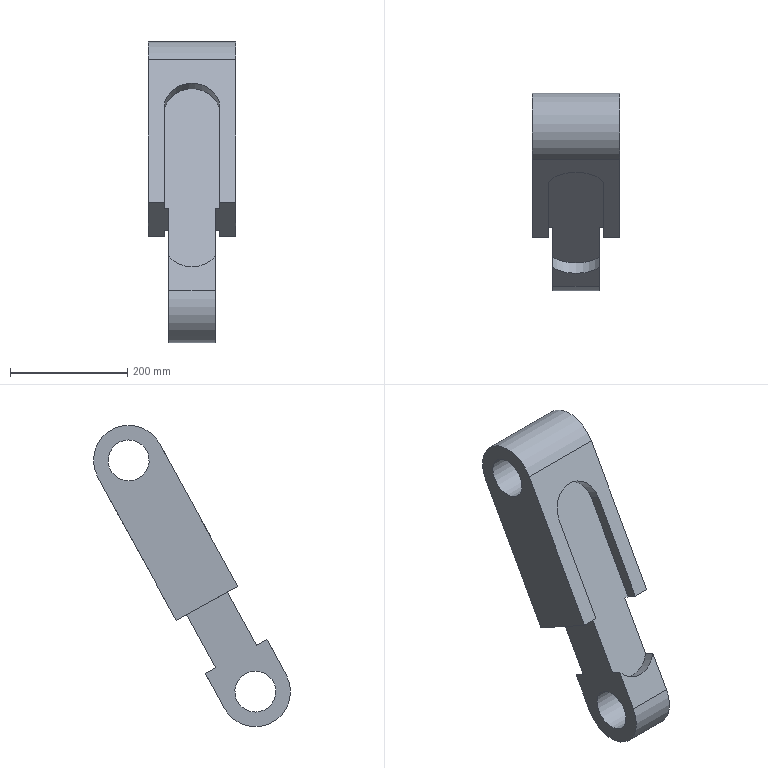Component | NX | UPPER_HYD_ROD | 1 solid | 28 faces | volume 5848426 mm3 | plane 20 | cylinder 8 | commonest cylinder face diameters 95 x4 120 x2 70 x2